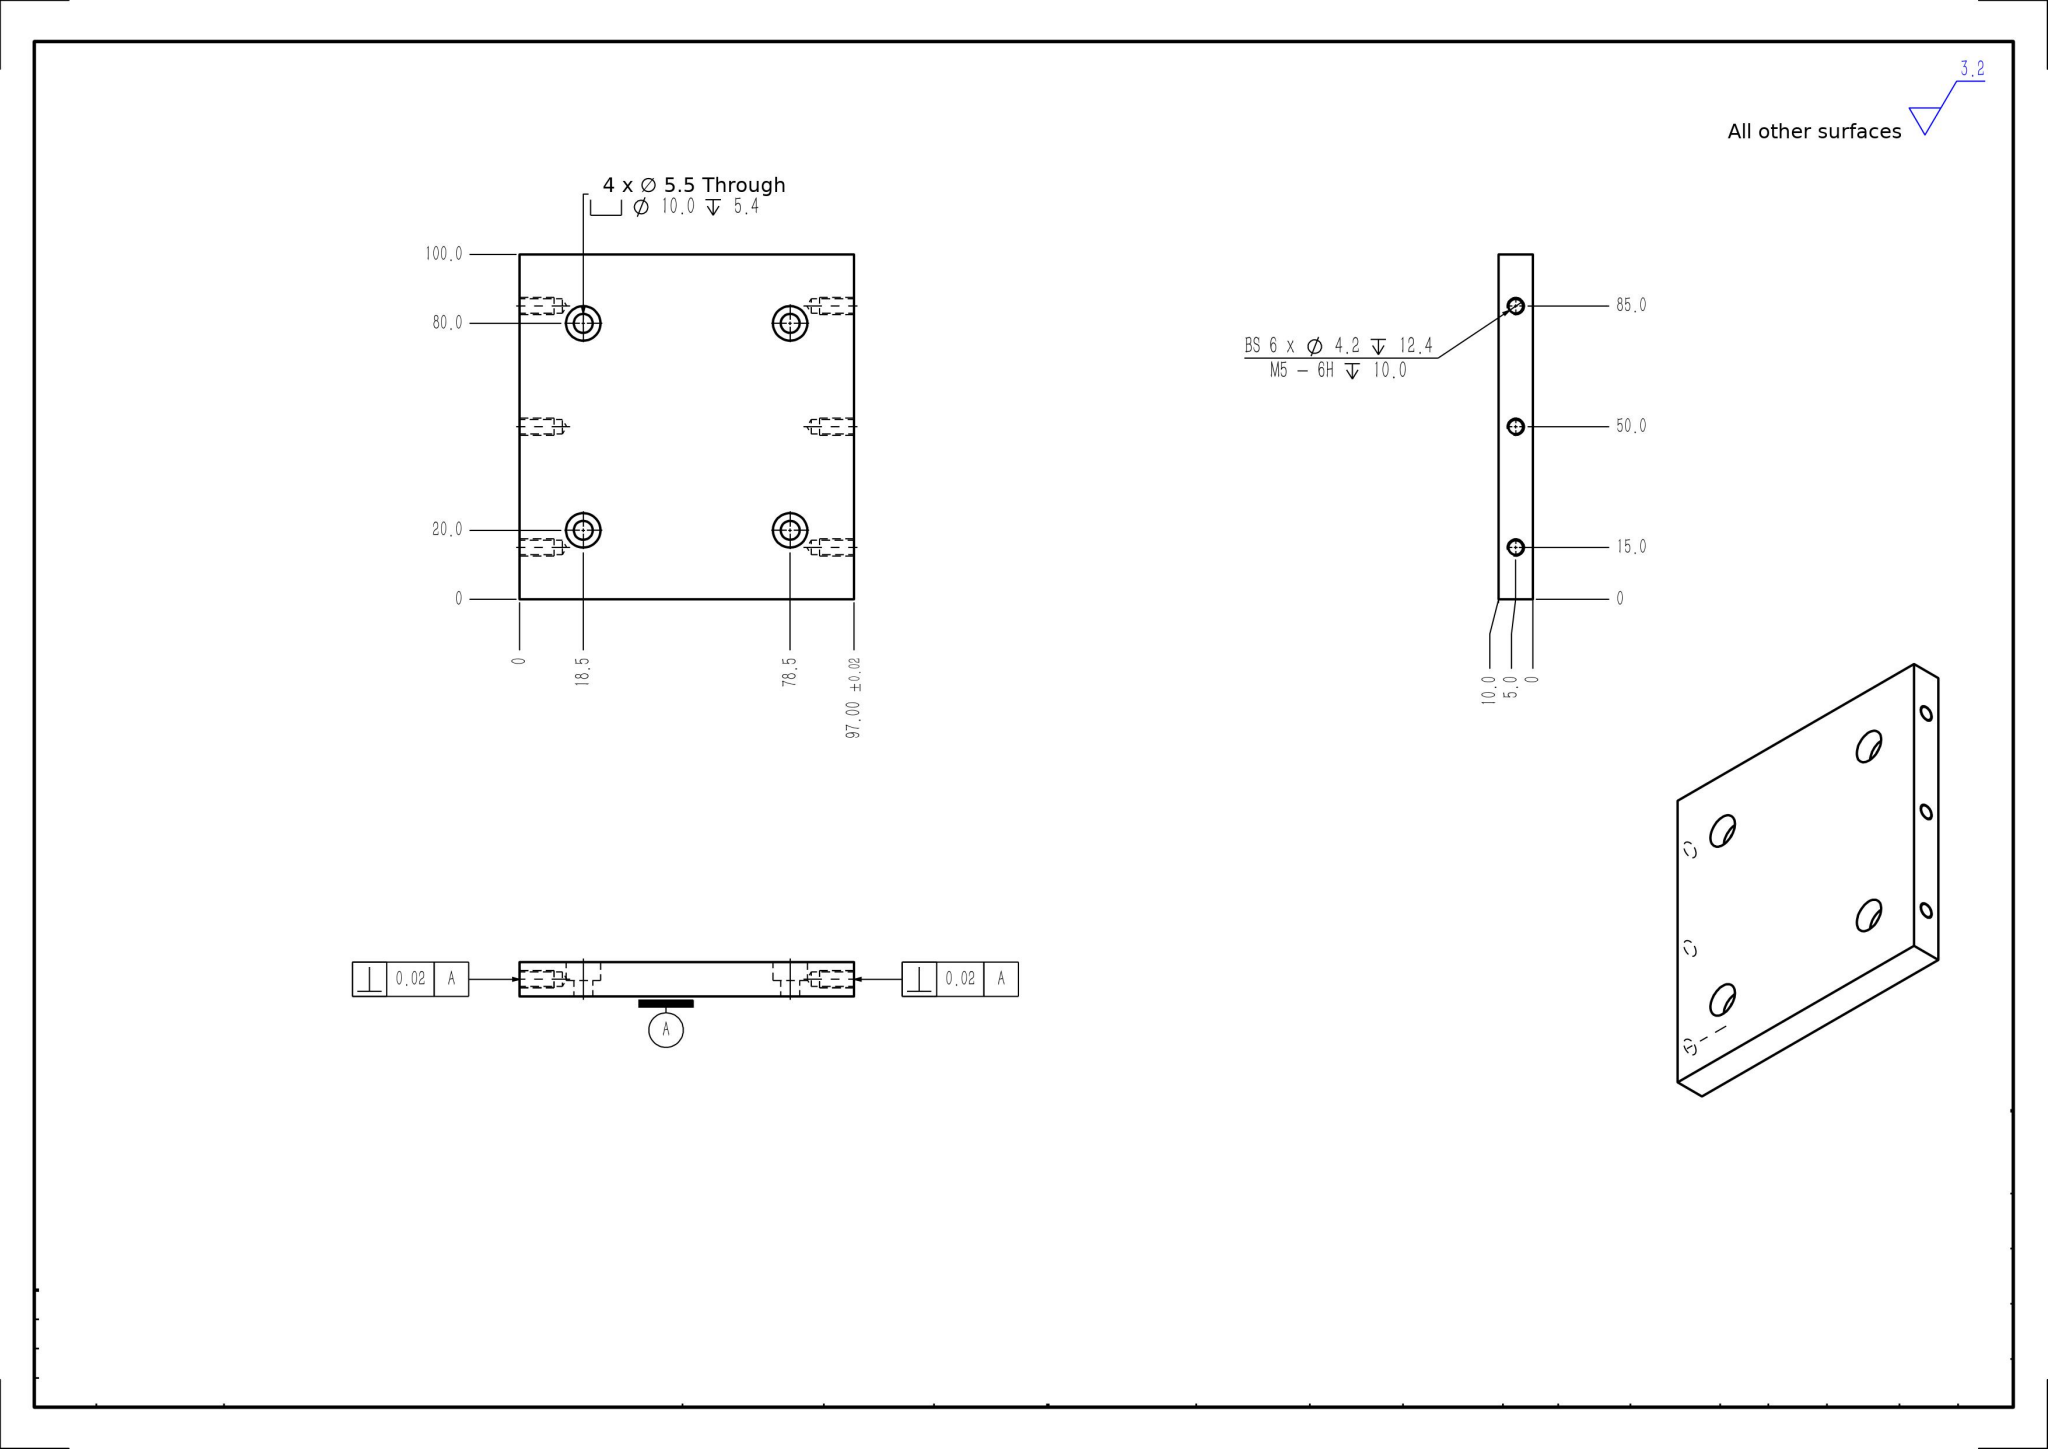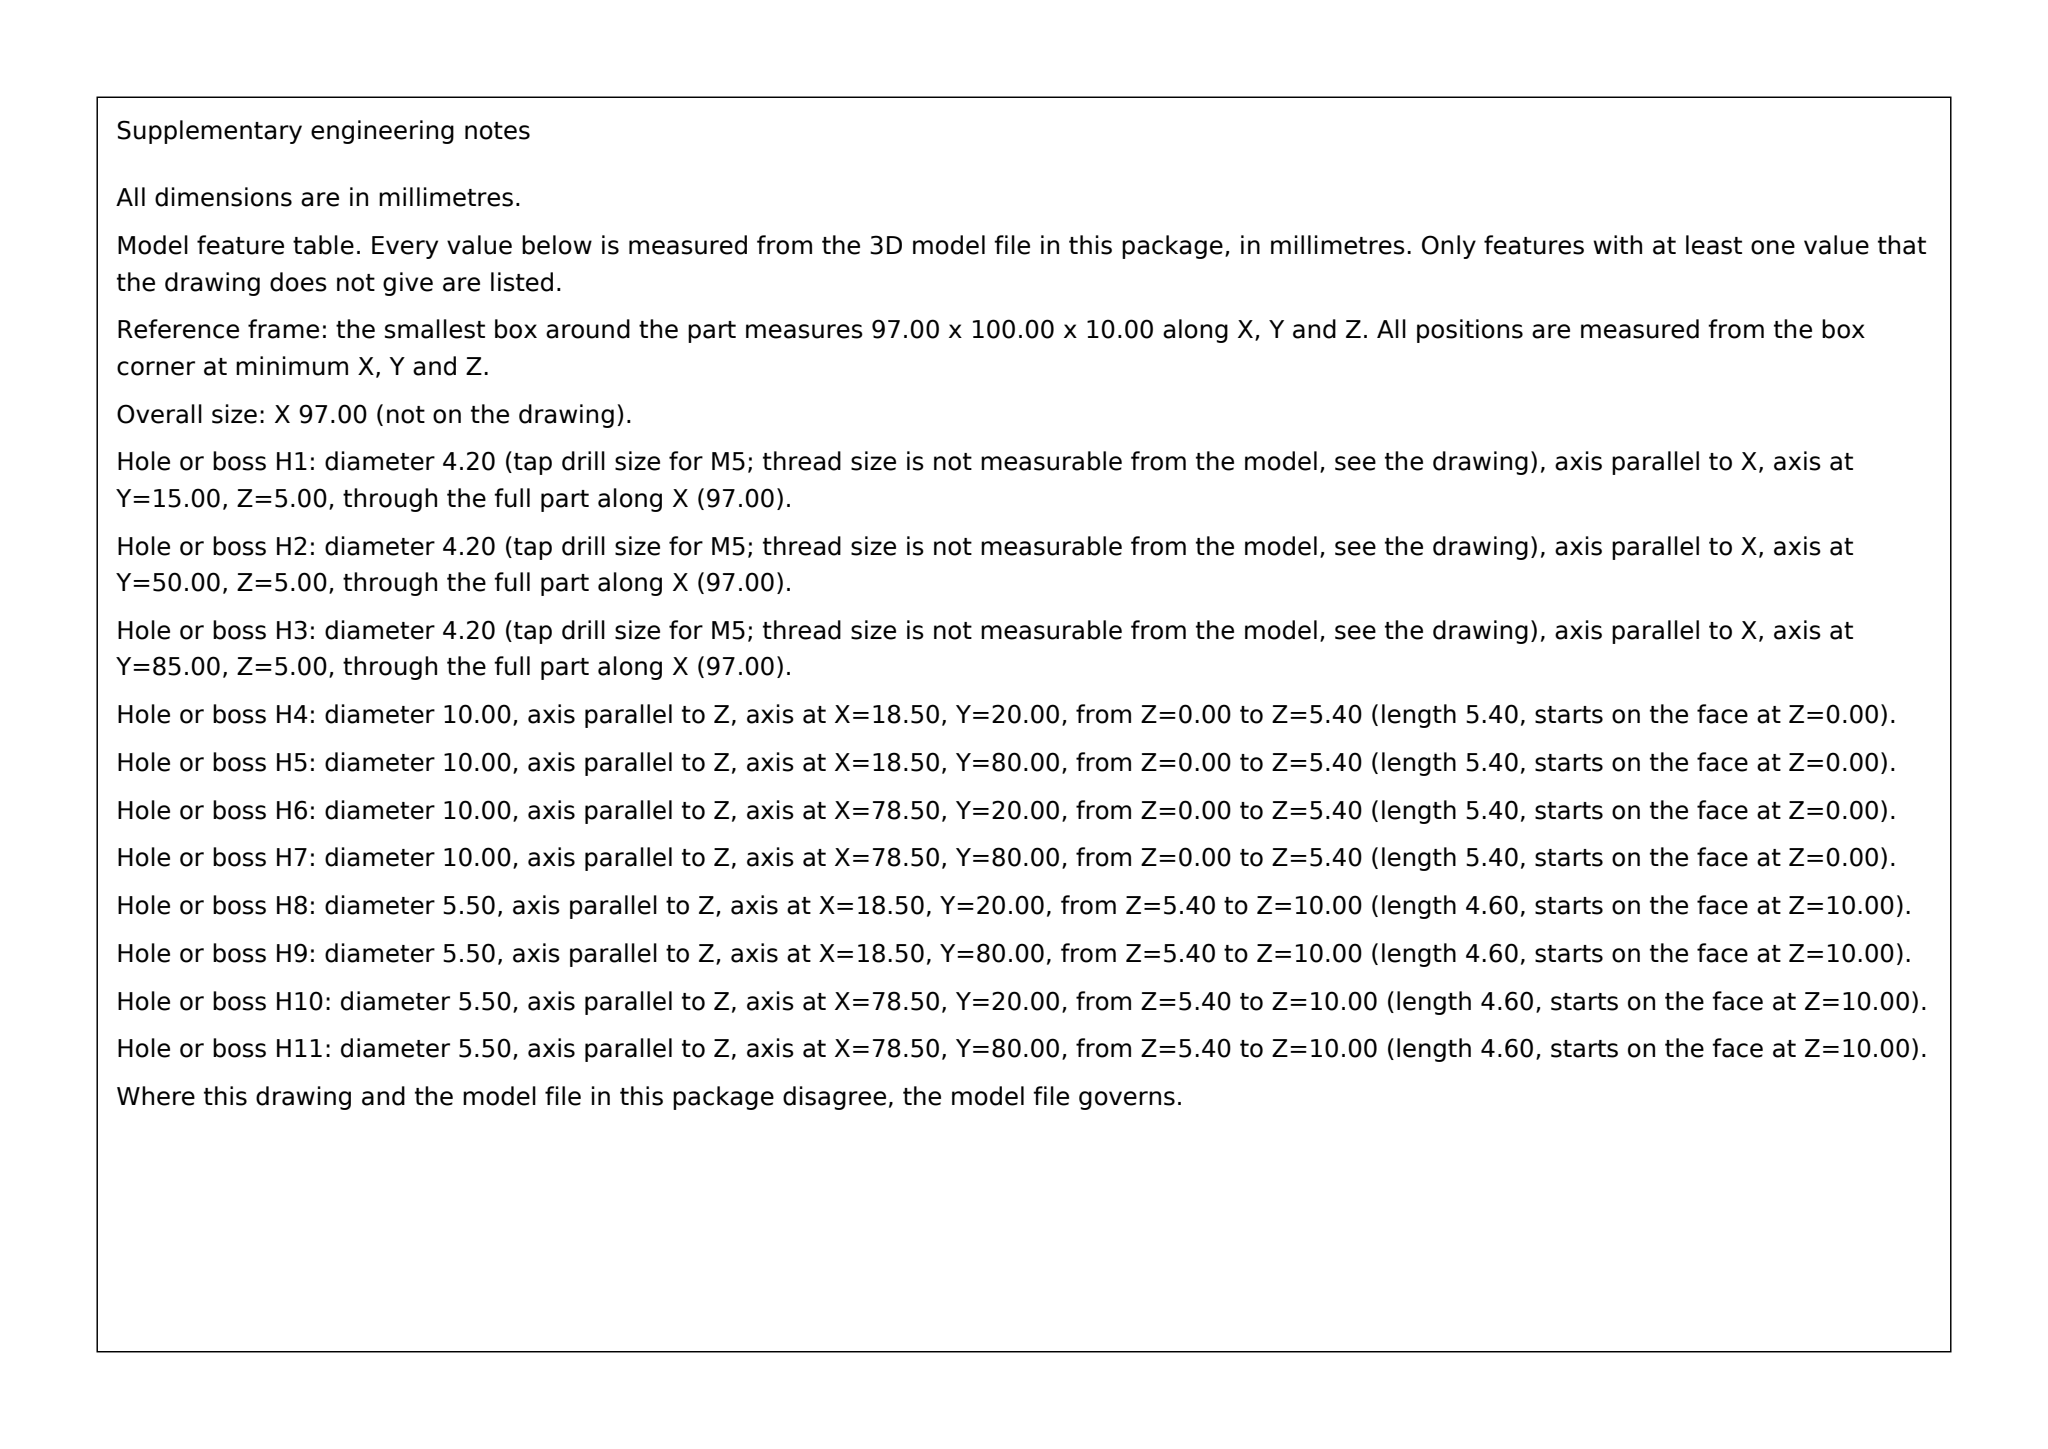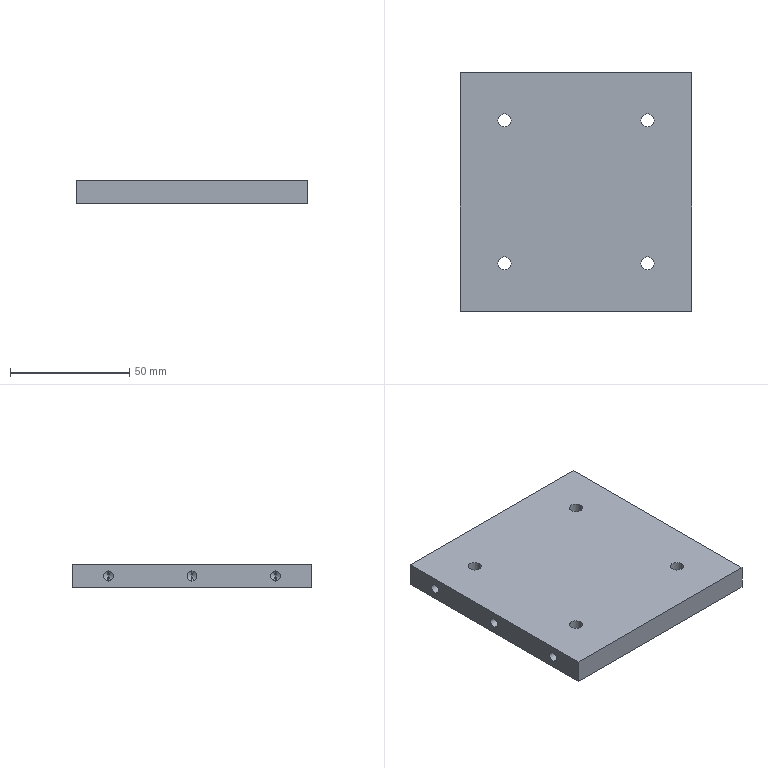Part | SolidWorks | mm | 1 solid | 50 faces | box 97 x 100 x 10 mm | volume 93801 mm3 | cylinder 28 | cone 12 | plane 10 | commonest cylinder face diameters 4.2 x12 10 x8 5.5 x8
build123d program:
from build123d import *

# Parameters (mm, degrees)
SKETCH1_W                                       = 97
SKETCH1_H                                       = 100
BOSS_EXTRUDE1_DEPTH                             = 5
M5_TAPPED_HOLE1_AT_2_COUNT                      = 2
M5_TAPPED_HOLE1_AT_2_PITCH                      = 35
M5_TAPPED_HOLE1_AT_3_COUNT                      = 2
M5_TAPPED_HOLE1_AT_3_PITCH                      = 35
M5_HEX_SOCKET_HEAD_CAP_SCREW_CBORE1_D           = 5.5
M5_HEX_SOCKET_HEAD_CAP_SCREW_CBORE1_CBORE_D     = 10
M5_HEX_SOCKET_HEAD_CAP_SCREW_CBORE1_CBORE_DEPTH = 5.4


with BuildPart() as part:
    # Sketch1 → Boss-Extrude1 (new, symmetric)
    with BuildSketch(Plane.XY):
        Rectangle(SKETCH1_W, SKETCH1_H)
    extrude(amount=BOSS_EXTRUDE1_DEPTH, both=True)

    # Sketch3 → M5 Tapped Hole1 (revolve, cut)
    with BuildSketch(Plane(origin=(-48.5, 0, 0), x_dir=(0, 0, 1), z_dir=(0, 1, 0))):
        Polygon((0, 0), (0, 13.662), (2.1, 12.4), (2.1, 0), align=None)
    m5_tapped_hole1 = revolve(axis=Axis((-54.85, 0, 0), (1, 0, 0)), mode=Mode.SUBTRACT)

    # M5 Tapped Hole1 at 2: M5 Tapped Hole1 ×2
    with Locations(*[(0, i * M5_TAPPED_HOLE1_AT_2_PITCH, 0) for i in range(1, M5_TAPPED_HOLE1_AT_2_COUNT)]):
        add(m5_tapped_hole1, mode=Mode.SUBTRACT)

    # M5 Tapped Hole1 at 3: M5 Tapped Hole1 ×2
    with Locations(*[(0, -i * M5_TAPPED_HOLE1_AT_3_PITCH, 0) for i in range(1, M5_TAPPED_HOLE1_AT_3_COUNT)]):
        add(m5_tapped_hole1, mode=Mode.SUBTRACT)

    # Mirror1: M5 Tapped Hole1 across plane
    add(m5_tapped_hole1.mirror(Plane(origin=(0, 0, 0), x_dir=(0, 0, 1), z_dir=(1, 0, 0))), mode=Mode.SUBTRACT)

    # Mirror1 copy 1 sketch → Mirror1 copy 1 (revolve, cut)
    with BuildSketch(Plane(origin=(48.5, 35, 0), x_dir=(0, 0, 1), z_dir=(0, 1, 0))):
        Polygon((0, 0), (0, -13.662), (2.1, -12.4), (2.1, 0), align=None)
    revolve(axis=Axis((54.85, 35, 0), (1, 0, 0)), mode=Mode.SUBTRACT)

    # Mirror1 copy 2 sketch → Mirror1 copy 2 (revolve, cut)
    with BuildSketch(Plane(origin=(48.5, -35, 0), x_dir=(0, 0, 1), z_dir=(0, 1, 0))):
        Polygon((0, 0), (0, -13.662), (2.1, -12.4), (2.1, 0), align=None)
    revolve(axis=Axis((54.85, -35, 0), (1, 0, 0)), mode=Mode.SUBTRACT)

    # M5 Hex Socket Head Cap Screw CBORE1 (through all)
    with Locations(Plane(origin=(0, 0, -5), x_dir=(-1, 0, 0), z_dir=(0, 0, -1))):
        with Locations((-30, 30), (30, 30), (-30, -30), (30, -30)):
            CounterBoreHole(M5_HEX_SOCKET_HEAD_CAP_SCREW_CBORE1_D / 2, M5_HEX_SOCKET_HEAD_CAP_SCREW_CBORE1_CBORE_D / 2, M5_HEX_SOCKET_HEAD_CAP_SCREW_CBORE1_CBORE_DEPTH)


solid = part.part